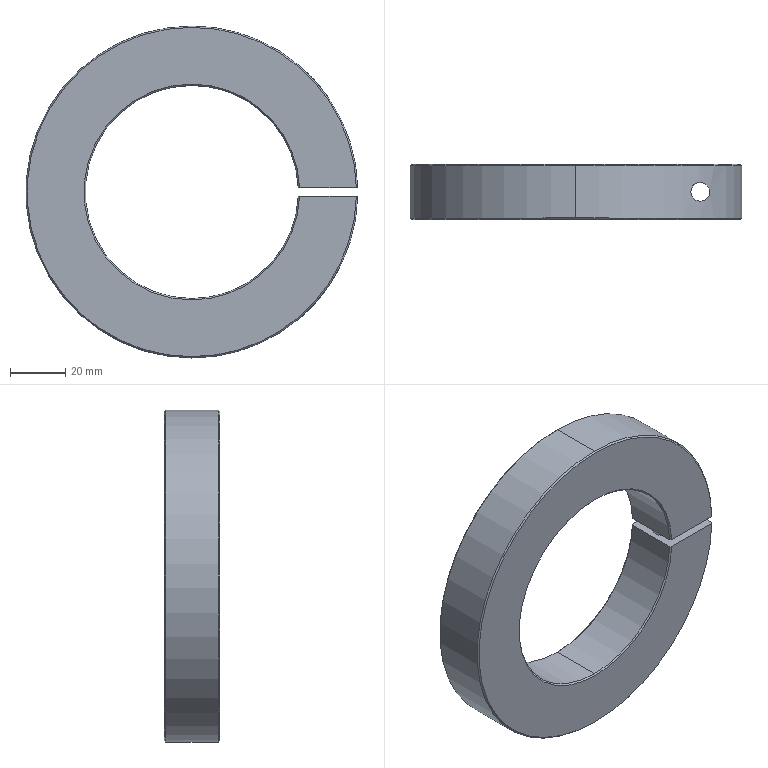Component | SolidWorks | 8TC-A15004-80-18A-1 | 1 solid | 29 faces | box 119.98 x 20 x 120 mm | volume 125088 mm3 | cylinder 12 | cone 12 | plane 5 | commonest cylinder face diameters 77 x3 120 x3 6.8 x2 9 x2 15 x2 | material Black POM
STEP:
#1=COLOUR_RGB('',0.7922,0.8196,0.9333);
#2=FILL_AREA_STYLE_COLOUR('',#1);
#3=FILL_AREA_STYLE('',(#2));
#4=SURFACE_STYLE_FILL_AREA(#3);
#5=SURFACE_SIDE_STYLE('',(#4));
#6=SURFACE_STYLE_USAGE(.BOTH.,#5);
#7=PRESENTATION_STYLE_ASSIGNMENT((#6));
#8=CARTESIAN_POINT('',(3.48,7.618,-28.131));
#9=VERTEX_POINT('',#8);
#10=CARTESIAN_POINT('',(3.213,7.618,-27.825));
#11=VERTEX_POINT('',#10);
#12=CARTESIAN_POINT('',(3.48,7.618,-28.131));
#13=CARTESIAN_POINT('',(3.48,7.613,-28.131));
#14=CARTESIAN_POINT('',(3.48,7.607,-28.131));
#15=CARTESIAN_POINT('',(3.479,7.596,-28.129));
#16=CARTESIAN_POINT('',(3.478,7.591,-28.128));
#17=CARTESIAN_POINT('',(3.475,7.58,-28.124));
#18=CARTESIAN_POINT('',(3.473,7.575,-28.122));
#19=CARTESIAN_POINT('',(3.47,7.566,-28.117));
#20=CARTESIAN_POINT('',(3.468,7.561,-28.115));
#21=CARTESIAN_POINT('',(3.463,7.553,-28.109));
#22=CARTESIAN_POINT('',(3.461,7.549,-28.106));
#23=CARTESIAN_POINT('',(3.456,7.541,-28.099));
#24=CARTESIAN_POINT('',(3.454,7.538,-28.096));
#25=CARTESIAN_POINT('',(3.445,7.528,-28.085));
#26=CARTESIAN_POINT('',(3.44,7.522,-28.078));
#27=CARTESIAN_POINT('',(3.421,7.506,-28.054));
#28=CARTESIAN_POINT('',(3.408,7.498,-28.038));
#29=CARTESIAN_POINT('',(3.388,7.491,-28.013));
#30=CARTESIAN_POINT('',(3.38,7.488,-28.004));
#31=CARTESIAN_POINT('',(3.366,7.486,-27.988));
#32=CARTESIAN_POINT('',(3.359,7.485,-27.979));
#33=CARTESIAN_POINT('',(3.344,7.484,-27.963));
#34=CARTESIAN_POINT('',(3.337,7.484,-27.954));
#35=CARTESIAN_POINT('',(3.322,7.486,-27.938));
#36=CARTESIAN_POINT('',(3.315,7.488,-27.93));
#37=CARTESIAN_POINT('',(3.3,7.492,-27.914));
#38=CARTESIAN_POINT('',(3.292,7.495,-27.906));
#39=CARTESIAN_POINT('',(3.278,7.503,-27.891));
#40=CARTESIAN_POINT('',(3.271,7.507,-27.883));
#41=CARTESIAN_POINT('',(3.257,7.518,-27.869));
#42=CARTESIAN_POINT('',(3.251,7.524,-27.863));
#43=CARTESIAN_POINT('',(3.238,7.538,-27.851));
#44=CARTESIAN_POINT('',(3.233,7.547,-27.845));
#45=CARTESIAN_POINT('',(3.223,7.565,-27.836));
#46=CARTESIAN_POINT('',(3.219,7.575,-27.832));
#47=CARTESIAN_POINT('',(3.214,7.596,-27.827));
#48=CARTESIAN_POINT('',(3.213,7.607,-27.825));
#49=CARTESIAN_POINT('',(3.213,7.618,-27.825));
#50=B_SPLINE_CURVE_WITH_KNOTS('',3,(#12,#13,#14,#15,#16,#17,#18,#19,#20,#21,#22,#23,#24,#25,#26,#27,#28,#29,#30,#31,#32,#33,#34,#35,#36,#37,#38,#39,#40,#41,#42,#43,#44,#45,#46,#47,#48,#49),.UNSPECIFIED.,.F.,.F.,(4,2,2,2,2,2,2,2,2,2,2,2,2,2,2,2,2,2,4),(0.01358,0.014,0.01443,0.01485,0.01527,0.0157,0.01612,0.01697,0.01867,0.01952,0.02037,0.02122,0.02206,0.02291,0.02376,0.02461,0.02546,0.02631,0.02716),.UNSPECIFIED.);
#51=EDGE_CURVE('',#9,#11,#50,.T.);
#52=ORIENTED_EDGE('',*,*,#51,.F.);
#53=CARTESIAN_POINT('',(3.48,7.618,-29.469));
#54=VERTEX_POINT('',#53);
#55=CARTESIAN_POINT('',(3.48,7.618,-29.469));
#56=DIRECTION('',(0.,0.,-1.));
#57=VECTOR('',#56,39.37);
#58=LINE('',#55,#57);
#59=EDGE_CURVE('',#9,#54,#58,.T.);
#60=ORIENTED_EDGE('',*,*,#59,.T.);
#61=CARTESIAN_POINT('',(3.213,7.618,-29.469));
#62=VERTEX_POINT('',#61);
#63=CARTESIAN_POINT('',(3.346,7.618,-29.469));
#64=DIRECTION('',(0.,0.,-1.));
#65=DIRECTION('',(-1.,0.,0.));
#66=AXIS2_PLACEMENT_3D('',#63,#64,#65);
#67=CIRCLE('',#66,0.1339);
#68=EDGE_CURVE('',#54,#62,#67,.T.);
#69=ORIENTED_EDGE('',*,*,#68,.T.);
#70=CARTESIAN_POINT('',(3.213,7.618,-29.469));
#71=DIRECTION('',(0.,0.,-1.));
#72=VECTOR('',#71,39.37);
#73=LINE('',#70,#72);
#74=EDGE_CURVE('',#11,#62,#73,.T.);
#75=ORIENTED_EDGE('',*,*,#74,.F.);
#76=EDGE_LOOP('',(#52,#60,#69,#75));
#77=FACE_OUTER_BOUND('',#76,.T.);
#78=CARTESIAN_POINT('',(3.346,7.618,-29.469));
#79=DIRECTION('',(0.,0.,-1.));
#80=DIRECTION('',(-1.,0.,0.));
#81=AXIS2_PLACEMENT_3D('',#78,#79,#80);
#82=CYLINDRICAL_SURFACE('',#81,0.1339);
#83=ADVANCED_FACE('',(#77),#82,.F.);
#84=CARTESIAN_POINT('',(1.575,7.244,-28.012));
#85=VERTEX_POINT('',#84);
#86=CARTESIAN_POINT('',(1.575,7.244,-31.043));
#87=VERTEX_POINT('',#86);
#88=CARTESIAN_POINT('',(1.575,7.244,-29.528));
#89=DIRECTION('',(0.,-1.,0.));
#90=DIRECTION('',(0.,0.,1.));
#91=AXIS2_PLACEMENT_3D('',#88,#89,#90);
#92=CIRCLE('',#91,1.516);
#93=EDGE_CURVE('',#85,#87,#92,.T.);
#94=ORIENTED_EDGE('',*,*,#93,.F.);
#95=CARTESIAN_POINT('',(1.575,7.224,-27.992));
#96=VERTEX_POINT('',#95);
#97=CARTESIAN_POINT('',(1.575,7.224,-27.992));
#98=DIRECTION('',(0.,-0.7071,0.7071));
#99=VECTOR('',#98,39.37);
#100=LINE('',#97,#99);
#101=EDGE_CURVE('',#85,#96,#100,.T.);
#102=ORIENTED_EDGE('',*,*,#101,.T.);
#103=CARTESIAN_POINT('',(1.575,7.224,-31.063));
#104=VERTEX_POINT('',#103);
#105=CARTESIAN_POINT('',(1.575,7.224,-29.528));
#106=DIRECTION('',(0.,1.,0.));
#107=DIRECTION('',(0.,0.,1.));
#108=AXIS2_PLACEMENT_3D('',#105,#106,#107);
#109=CIRCLE('',#108,1.535);
#110=EDGE_CURVE('',#104,#96,#109,.T.);
#111=ORIENTED_EDGE('',*,*,#110,.F.);
#112=CARTESIAN_POINT('',(1.575,7.224,-31.063));
#113=DIRECTION('',(0.,-0.7071,-0.7071));
#114=VECTOR('',#113,39.37);
#115=LINE('',#112,#114);
#116=EDGE_CURVE('',#87,#104,#115,.T.);
#117=ORIENTED_EDGE('',*,*,#116,.F.);
#118=EDGE_LOOP('',(#94,#102,#111,#117));
#119=FACE_OUTER_BOUND('',#118,.T.);
#120=CARTESIAN_POINT('',(1.575,7.224,-29.528));
#121=DIRECTION('',(0.,-1.,0.));
#122=DIRECTION('',(0.,0.,-1.));
#123=AXIS2_PLACEMENT_3D('',#120,#121,#122);
#124=CONICAL_SURFACE('',#123,1.535,0.7854);
#125=ADVANCED_FACE('',(#119),#124,.F.);
#126=CARTESIAN_POINT('',(3.089,7.244,-29.587));
#127=VERTEX_POINT('',#126);
#128=CARTESIAN_POINT('',(1.575,7.244,-29.528));
#129=DIRECTION('',(0.,-1.,0.));
#130=DIRECTION('',(0.,0.,1.));
#131=AXIS2_PLACEMENT_3D('',#128,#129,#130);
#132=CIRCLE('',#131,1.516);
#133=EDGE_CURVE('',#87,#127,#132,.T.);
#134=ORIENTED_EDGE('',*,*,#133,.F.);
#135=ORIENTED_EDGE('',*,*,#116,.T.);
#136=CARTESIAN_POINT('',(3.109,7.224,-29.587));
#137=VERTEX_POINT('',#136);
#138=CARTESIAN_POINT('',(1.575,7.224,-29.528));
#139=DIRECTION('',(0.,1.,0.));
#140=DIRECTION('',(0.,0.,1.));
#141=AXIS2_PLACEMENT_3D('',#138,#139,#140);
#142=CIRCLE('',#141,1.535);
#143=EDGE_CURVE('',#137,#104,#142,.T.);
#144=ORIENTED_EDGE('',*,*,#143,.F.);
#145=CARTESIAN_POINT('',(3.089,7.244,-29.587));
#146=CARTESIAN_POINT('',(3.096,7.238,-29.587));
#147=CARTESIAN_POINT('',(3.103,7.231,-29.587));
#148=CARTESIAN_POINT('',(3.109,7.224,-29.587));
#149=B_SPLINE_CURVE_WITH_KNOTS('',3,(#145,#146,#147,#148),.UNSPECIFIED.,.F.,.F.,(4,4),(0.,0.0007074),.UNSPECIFIED.);
#150=EDGE_CURVE('',#127,#137,#149,.T.);
#151=ORIENTED_EDGE('',*,*,#150,.F.);
#152=EDGE_LOOP('',(#134,#135,#144,#151));
#153=FACE_OUTER_BOUND('',#152,.T.);
#154=CARTESIAN_POINT('',(1.575,7.224,-29.528));
#155=DIRECTION('',(0.,-1.,0.));
#156=DIRECTION('',(0.,0.,-1.));
#157=AXIS2_PLACEMENT_3D('',#154,#155,#156);
#158=CONICAL_SURFACE('',#157,1.535,0.7854);
#159=ADVANCED_FACE('',(#153),#158,.F.);
#160=CARTESIAN_POINT('',(1.575,7.224,-31.87));
#161=VERTEX_POINT('',#160);
#162=CARTESIAN_POINT('',(3.917,7.224,-29.587));
#163=VERTEX_POINT('',#162);
#164=CARTESIAN_POINT('',(1.575,7.224,-29.528));
#165=DIRECTION('',(0.,-1.,0.));
#166=DIRECTION('',(-0.,0.,1.));
#167=AXIS2_PLACEMENT_3D('',#164,#165,#166);
#168=CIRCLE('',#167,2.343);
#169=EDGE_CURVE('',#161,#163,#168,.T.);
#170=ORIENTED_EDGE('',*,*,#169,.F.);
#171=CARTESIAN_POINT('',(1.575,7.244,-31.89));
#172=VERTEX_POINT('',#171);
#173=CARTESIAN_POINT('',(1.575,7.244,-31.89));
#174=DIRECTION('',(0.,0.7071,-0.7071));
#175=VECTOR('',#174,39.37);
#176=LINE('',#173,#175);
#177=EDGE_CURVE('',#161,#172,#176,.T.);
#178=ORIENTED_EDGE('',*,*,#177,.T.);
#179=CARTESIAN_POINT('',(3.936,7.244,-29.587));
#180=VERTEX_POINT('',#179);
#181=CARTESIAN_POINT('',(1.575,7.244,-29.528));
#182=DIRECTION('',(0.,1.,0.));
#183=DIRECTION('',(0.,0.,1.));
#184=AXIS2_PLACEMENT_3D('',#181,#182,#183);
#185=CIRCLE('',#184,2.362);
#186=EDGE_CURVE('',#180,#172,#185,.T.);
#187=ORIENTED_EDGE('',*,*,#186,.F.);
#188=CARTESIAN_POINT('',(3.917,7.224,-29.587));
#189=CARTESIAN_POINT('',(3.923,7.231,-29.587));
#190=CARTESIAN_POINT('',(3.93,7.238,-29.587));
#191=CARTESIAN_POINT('',(3.936,7.244,-29.587));
#192=B_SPLINE_CURVE_WITH_KNOTS('',3,(#188,#189,#190,#191),.UNSPECIFIED.,.F.,.F.,(4,4),(0.,0.0007072),.UNSPECIFIED.);
#193=EDGE_CURVE('',#163,#180,#192,.T.);
#194=ORIENTED_EDGE('',*,*,#193,.F.);
#195=EDGE_LOOP('',(#170,#178,#187,#194));
#196=FACE_OUTER_BOUND('',#195,.T.);
#197=CARTESIAN_POINT('',(1.575,7.244,-29.528));
#198=DIRECTION('',(0.,1.,0.));
#199=DIRECTION('',(0.,0.,1.));
#200=AXIS2_PLACEMENT_3D('',#197,#198,#199);
#201=CONICAL_SURFACE('',#200,2.362,0.7854);
#202=ADVANCED_FACE('',(#196),#201,.T.);
#203=ORIENTED_EDGE('',*,*,#177,.F.);
#204=CARTESIAN_POINT('',(1.575,7.224,-27.185));
#205=VERTEX_POINT('',#204);
#206=CARTESIAN_POINT('',(1.575,7.224,-29.528));
#207=DIRECTION('',(0.,-1.,0.));
#208=DIRECTION('',(0.,0.,1.));
#209=AXIS2_PLACEMENT_3D('',#206,#207,#208);
#210=CIRCLE('',#209,2.343);
#211=EDGE_CURVE('',#205,#161,#210,.T.);
#212=ORIENTED_EDGE('',*,*,#211,.F.);
#213=CARTESIAN_POINT('',(1.575,7.244,-27.165));
#214=VERTEX_POINT('',#213);
#215=CARTESIAN_POINT('',(1.575,7.244,-27.165));
#216=DIRECTION('',(0.,0.7071,0.7071));
#217=VECTOR('',#216,39.37);
#218=LINE('',#215,#217);
#219=EDGE_CURVE('',#205,#214,#218,.T.);
#220=ORIENTED_EDGE('',*,*,#219,.T.);
#221=CARTESIAN_POINT('',(1.575,7.244,-29.528));
#222=DIRECTION('',(0.,1.,0.));
#223=DIRECTION('',(0.,0.,1.));
#224=AXIS2_PLACEMENT_3D('',#221,#222,#223);
#225=CIRCLE('',#224,2.362);
#226=EDGE_CURVE('',#172,#214,#225,.T.);
#227=ORIENTED_EDGE('',*,*,#226,.F.);
#228=EDGE_LOOP('',(#203,#212,#220,#227));
#229=FACE_OUTER_BOUND('',#228,.T.);
#230=CARTESIAN_POINT('',(1.575,7.244,-29.528));
#231=DIRECTION('',(0.,1.,0.));
#232=DIRECTION('',(0.,0.,1.));
#233=AXIS2_PLACEMENT_3D('',#230,#231,#232);
#234=CONICAL_SURFACE('',#233,2.362,0.7854);
#235=ADVANCED_FACE('',(#229),#234,.T.);
#236=CARTESIAN_POINT('',(1.575,8.012,-27.185));
#237=VERTEX_POINT('',#236);
#238=CARTESIAN_POINT('',(3.917,8.012,-29.469));
#239=VERTEX_POINT('',#238);
#240=CARTESIAN_POINT('',(1.575,8.012,-29.528));
#241=DIRECTION('',(0.,1.,0.));
#242=DIRECTION('',(0.,0.,1.));
#243=AXIS2_PLACEMENT_3D('',#240,#241,#242);
#244=CIRCLE('',#243,2.343);
#245=EDGE_CURVE('',#237,#239,#244,.T.);
#246=ORIENTED_EDGE('',*,*,#245,.F.);
#247=CARTESIAN_POINT('',(1.575,7.992,-27.165));
#248=VERTEX_POINT('',#247);
#249=CARTESIAN_POINT('',(1.575,8.012,-27.185));
#250=DIRECTION('',(0.,-0.7071,0.7071));
#251=VECTOR('',#250,39.37);
#252=LINE('',#249,#251);
#253=EDGE_CURVE('',#237,#248,#252,.T.);
#254=ORIENTED_EDGE('',*,*,#253,.T.);
#255=CARTESIAN_POINT('',(3.936,7.992,-29.469));
#256=VERTEX_POINT('',#255);
#257=CARTESIAN_POINT('',(1.575,7.992,-29.528));
#258=DIRECTION('',(0.,-1.,0.));
#259=DIRECTION('',(-0.,0.,1.));
#260=AXIS2_PLACEMENT_3D('',#257,#258,#259);
#261=CIRCLE('',#260,2.362);
#262=EDGE_CURVE('',#256,#248,#261,.T.);
#263=ORIENTED_EDGE('',*,*,#262,.F.);
#264=CARTESIAN_POINT('',(3.917,8.012,-29.469));
#265=CARTESIAN_POINT('',(3.923,8.005,-29.469));
#266=CARTESIAN_POINT('',(3.93,7.999,-29.469));
#267=CARTESIAN_POINT('',(3.936,7.992,-29.469));
#268=B_SPLINE_CURVE_WITH_KNOTS('',3,(#264,#265,#266,#267),.UNSPECIFIED.,.F.,.F.,(4,4),(0.,0.0007072),.UNSPECIFIED.);
#269=EDGE_CURVE('',#239,#256,#268,.T.);
#270=ORIENTED_EDGE('',*,*,#269,.F.);
#271=EDGE_LOOP('',(#246,#254,#263,#270));
#272=FACE_OUTER_BOUND('',#271,.T.);
#273=CARTESIAN_POINT('',(1.575,8.012,-29.528));
#274=DIRECTION('',(0.,-1.,0.));
#275=DIRECTION('',(0.,0.,-1.));
#276=AXIS2_PLACEMENT_3D('',#273,#274,#275);
#277=CONICAL_SURFACE('',#276,2.343,0.7854);
#278=ADVANCED_FACE('',(#272),#277,.T.);
#279=ORIENTED_EDGE('',*,*,#253,.F.);
#280=CARTESIAN_POINT('',(1.575,8.012,-31.87));
#281=VERTEX_POINT('',#280);
#282=CARTESIAN_POINT('',(1.575,8.012,-29.528));
#283=DIRECTION('',(0.,1.,0.));
#284=DIRECTION('',(0.,0.,1.));
#285=AXIS2_PLACEMENT_3D('',#282,#283,#284);
#286=CIRCLE('',#285,2.343);
#287=EDGE_CURVE('',#281,#237,#286,.T.);
#288=ORIENTED_EDGE('',*,*,#287,.F.);
#289=CARTESIAN_POINT('',(1.575,7.992,-31.89));
#290=VERTEX_POINT('',#289);
#291=CARTESIAN_POINT('',(1.575,8.012,-31.87));
#292=DIRECTION('',(0.,-0.7071,-0.7071));
#293=VECTOR('',#292,39.37);
#294=LINE('',#291,#293);
#295=EDGE_CURVE('',#281,#290,#294,.T.);
#296=ORIENTED_EDGE('',*,*,#295,.T.);
#297=CARTESIAN_POINT('',(1.575,7.992,-29.528));
#298=DIRECTION('',(0.,-1.,0.));
#299=DIRECTION('',(0.,0.,1.));
#300=AXIS2_PLACEMENT_3D('',#297,#298,#299);
#301=CIRCLE('',#300,2.362);
#302=EDGE_CURVE('',#248,#290,#301,.T.);
#303=ORIENTED_EDGE('',*,*,#302,.F.);
#304=EDGE_LOOP('',(#279,#288,#296,#303));
#305=FACE_OUTER_BOUND('',#304,.T.);
#306=CARTESIAN_POINT('',(1.575,8.012,-29.528));
#307=DIRECTION('',(0.,-1.,0.));
#308=DIRECTION('',(0.,0.,-1.));
#309=AXIS2_PLACEMENT_3D('',#306,#307,#308);
#310=CONICAL_SURFACE('',#309,2.343,0.7854);
#311=ADVANCED_FACE('',(#305),#310,.T.);
#312=CARTESIAN_POINT('',(1.575,7.992,-31.043));
#313=VERTEX_POINT('',#312);
#314=CARTESIAN_POINT('',(1.575,7.992,-28.012));
#315=VERTEX_POINT('',#314);
#316=CARTESIAN_POINT('',(1.575,7.992,-29.528));
#317=DIRECTION('',(0.,1.,0.));
#318=DIRECTION('',(0.,0.,1.));
#319=AXIS2_PLACEMENT_3D('',#316,#317,#318);
#320=CIRCLE('',#319,1.516);
#321=EDGE_CURVE('',#313,#315,#320,.T.);
#322=ORIENTED_EDGE('',*,*,#321,.F.);
#323=CARTESIAN_POINT('',(1.575,8.012,-31.063));
#324=VERTEX_POINT('',#323);
#325=CARTESIAN_POINT('',(1.575,7.992,-31.043));
#326=DIRECTION('',(0.,0.7071,-0.7071));
#327=VECTOR('',#326,39.37);
#328=LINE('',#325,#327);
#329=EDGE_CURVE('',#313,#324,#328,.T.);
#330=ORIENTED_EDGE('',*,*,#329,.T.);
#331=CARTESIAN_POINT('',(1.575,8.012,-27.992));
#332=VERTEX_POINT('',#331);
#333=CARTESIAN_POINT('',(1.575,8.012,-29.528));
#334=DIRECTION('',(0.,-1.,0.));
#335=DIRECTION('',(0.,0.,1.));
#336=AXIS2_PLACEMENT_3D('',#333,#334,#335);
#337=CIRCLE('',#336,1.535);
#338=EDGE_CURVE('',#332,#324,#337,.T.);
#339=ORIENTED_EDGE('',*,*,#338,.F.);
#340=CARTESIAN_POINT('',(1.575,7.992,-28.012));
#341=DIRECTION('',(0.,0.7071,0.7071));
#342=VECTOR('',#341,39.37);
#343=LINE('',#340,#342);
#344=EDGE_CURVE('',#315,#332,#343,.T.);
#345=ORIENTED_EDGE('',*,*,#344,.F.);
#346=EDGE_LOOP('',(#322,#330,#339,#345));
#347=FACE_OUTER_BOUND('',#346,.T.);
#348=CARTESIAN_POINT('',(1.575,7.992,-29.528));
#349=DIRECTION('',(0.,1.,0.));
#350=DIRECTION('',(0.,0.,1.));
#351=AXIS2_PLACEMENT_3D('',#348,#349,#350);
#352=CONICAL_SURFACE('',#351,1.516,0.7854);
#353=ADVANCED_FACE('',(#347),#352,.F.);
#354=CARTESIAN_POINT('',(3.089,7.992,-29.469));
#355=VERTEX_POINT('',#354);
#356=CARTESIAN_POINT('',(1.575,7.992,-29.528));
#357=DIRECTION('',(0.,1.,0.));
#358=DIRECTION('',(0.,0.,1.));
#359=AXIS2_PLACEMENT_3D('',#356,#357,#358);
#360=CIRCLE('',#359,1.516);
#361=EDGE_CURVE('',#315,#355,#360,.T.);
#362=ORIENTED_EDGE('',*,*,#361,.F.);
#363=ORIENTED_EDGE('',*,*,#344,.T.);
#364=CARTESIAN_POINT('',(3.109,8.012,-29.469));
#365=VERTEX_POINT('',#364);
#366=CARTESIAN_POINT('',(1.575,8.012,-29.528));
#367=DIRECTION('',(0.,-1.,0.));
#368=DIRECTION('',(-0.,0.,1.));
#369=AXIS2_PLACEMENT_3D('',#366,#367,#368);
#370=CIRCLE('',#369,1.535);
#371=EDGE_CURVE('',#365,#332,#370,.T.);
#372=ORIENTED_EDGE('',*,*,#371,.F.);
#373=CARTESIAN_POINT('',(3.089,7.992,-29.469));
#374=CARTESIAN_POINT('',(3.096,7.999,-29.469));
#375=CARTESIAN_POINT('',(3.103,8.005,-29.469));
#376=CARTESIAN_POINT('',(3.109,8.012,-29.469));
#377=B_SPLINE_CURVE_WITH_KNOTS('',3,(#373,#374,#375,#376),.UNSPECIFIED.,.F.,.F.,(4,4),(0.,0.0007074),.UNSPECIFIED.);
#378=EDGE_CURVE('',#355,#365,#377,.T.);
#379=ORIENTED_EDGE('',*,*,#378,.F.);
#380=EDGE_LOOP('',(#362,#363,#372,#379));
#381=FACE_OUTER_BOUND('',#380,.T.);
#382=CARTESIAN_POINT('',(1.575,7.992,-29.528));
#383=DIRECTION('',(0.,1.,0.));
#384=DIRECTION('',(0.,0.,1.));
#385=AXIS2_PLACEMENT_3D('',#382,#383,#384);
#386=CONICAL_SURFACE('',#385,1.516,0.7854);
#387=ADVANCED_FACE('',(#381),#386,.F.);
#388=CARTESIAN_POINT('',(3.169,7.618,-29.587));
#389=VERTEX_POINT('',#388);
#390=CARTESIAN_POINT('',(3.524,7.618,-29.587));
#391=VERTEX_POINT('',#390);
#392=CARTESIAN_POINT('',(3.346,7.618,-29.587));
#393=DIRECTION('',(-0.,0.,1.));
#394=DIRECTION('',(-1.,0.,0.));
#395=AXIS2_PLACEMENT_3D('',#392,#393,#394);
#396=CIRCLE('',#395,0.1772);
#397=EDGE_CURVE('',#389,#391,#396,.T.);
#398=ORIENTED_EDGE('',*,*,#397,.T.);
#399=CARTESIAN_POINT('',(3.524,7.618,-30.118));
#400=VERTEX_POINT('',#399);
#401=CARTESIAN_POINT('',(3.524,7.618,-31.496));
#402=DIRECTION('',(0.,0.,-1.));
#403=VECTOR('',#402,39.37);
#404=LINE('',#401,#403);
#405=EDGE_CURVE('',#391,#400,#404,.T.);
#406=ORIENTED_EDGE('',*,*,#405,.T.);
#407=CARTESIAN_POINT('',(3.169,7.618,-30.118));
#408=VERTEX_POINT('',#407);
#409=CARTESIAN_POINT('',(3.346,7.618,-30.118));
#410=DIRECTION('',(0.,0.,-1.));
#411=DIRECTION('',(-1.,0.,0.));
#412=AXIS2_PLACEMENT_3D('',#409,#410,#411);
#413=CIRCLE('',#412,0.1772);
#414=EDGE_CURVE('',#400,#408,#413,.T.);
#415=ORIENTED_EDGE('',*,*,#414,.T.);
#416=CARTESIAN_POINT('',(3.169,7.618,-31.496));
#417=DIRECTION('',(0.,0.,-1.));
#418=VECTOR('',#417,39.37);
#419=LINE('',#416,#418);
#420=EDGE_CURVE('',#389,#408,#419,.T.);
#421=ORIENTED_EDGE('',*,*,#420,.F.);
#422=EDGE_LOOP('',(#398,#406,#415,#421));
#423=FACE_OUTER_BOUND('',#422,.T.);
#424=CARTESIAN_POINT('',(3.346,7.618,-31.496));
#425=DIRECTION('',(0.,0.,-1.));
#426=DIRECTION('',(-1.,0.,0.));
#427=AXIS2_PLACEMENT_3D('',#424,#425,#426);
#428=CYLINDRICAL_SURFACE('',#427,0.1772);
#429=ADVANCED_FACE('',(#423),#428,.F.);
#430=CARTESIAN_POINT('',(3.642,7.618,-30.118));
#431=VERTEX_POINT('',#430);
#432=CARTESIAN_POINT('',(3.051,7.618,-30.118));
#433=VERTEX_POINT('',#432);
#434=CARTESIAN_POINT('',(3.346,7.618,-30.118));
#435=DIRECTION('',(0.,0.,-1.));
#436=DIRECTION('',(-1.,0.,0.));
#437=AXIS2_PLACEMENT_3D('',#434,#435,#436);
#438=CIRCLE('',#437,0.2953);
#439=EDGE_CURVE('',#431,#433,#438,.T.);
#440=ORIENTED_EDGE('',*,*,#439,.F.);
#441=CARTESIAN_POINT('',(3.642,7.618,-30.671));
#442=VERTEX_POINT('',#441);
#443=CARTESIAN_POINT('',(3.642,7.618,-31.496));
#444=DIRECTION('',(0.,0.,-1.));
#445=VECTOR('',#444,39.37);
#446=LINE('',#443,#445);
#447=EDGE_CURVE('',#431,#442,#446,.T.);
#448=ORIENTED_EDGE('',*,*,#447,.T.);
#449=CARTESIAN_POINT('',(3.051,7.618,-31.372));
#450=VERTEX_POINT('',#449);
#451=CARTESIAN_POINT('',(3.051,7.618,-31.372));
#452=CARTESIAN_POINT('',(3.051,7.593,-31.372));
#453=CARTESIAN_POINT('',(3.054,7.568,-31.369));
#454=CARTESIAN_POINT('',(3.064,7.532,-31.361));
#455=CARTESIAN_POINT('',(3.067,7.521,-31.358));
#456=CARTESIAN_POINT('',(3.076,7.498,-31.351));
#457=CARTESIAN_POINT('',(3.081,7.488,-31.347));
#458=CARTESIAN_POINT('',(3.092,7.467,-31.338));
#459=CARTESIAN_POINT('',(3.099,7.457,-31.333));
#460=CARTESIAN_POINT('',(3.112,7.439,-31.322));
#461=CARTESIAN_POINT('',(3.118,7.43,-31.316));
#462=CARTESIAN_POINT('',(3.133,7.414,-31.303));
#463=CARTESIAN_POINT('',(3.14,7.406,-31.296));
#464=CARTESIAN_POINT('',(3.156,7.392,-31.283));
#465=CARTESIAN_POINT('',(3.164,7.386,-31.275));
#466=CARTESIAN_POINT('',(3.188,7.368,-31.253));
#467=CARTESIAN_POINT('',(3.205,7.358,-31.237));
#468=CARTESIAN_POINT('',(3.23,7.346,-31.213));
#469=CARTESIAN_POINT('',(3.239,7.343,-31.204));
#470=CARTESIAN_POINT('',(3.256,7.337,-31.187));
#471=CARTESIAN_POINT('',(3.265,7.334,-31.178));
#472=CARTESIAN_POINT('',(3.29,7.328,-31.152));
#473=CARTESIAN_POINT('',(3.307,7.325,-31.134));
#474=CARTESIAN_POINT('',(3.341,7.322,-31.097));
#475=CARTESIAN_POINT('',(3.357,7.323,-31.078));
#476=CARTESIAN_POINT('',(3.406,7.327,-31.021));
#477=CARTESIAN_POINT('',(3.436,7.335,-30.983));
#478=CARTESIAN_POINT('',(3.479,7.354,-30.925));
#479=CARTESIAN_POINT('',(3.493,7.361,-30.906));
#480=CARTESIAN_POINT('',(3.52,7.379,-30.867));
#481=CARTESIAN_POINT('',(3.533,7.389,-30.849));
#482=CARTESIAN_POINT('',(3.558,7.411,-30.811));
#483=CARTESIAN_POINT('',(3.569,7.424,-30.793));
#484=CARTESIAN_POINT('',(3.586,7.445,-30.767));
#485=CARTESIAN_POINT('',(3.591,7.452,-30.758));
#486=CARTESIAN_POINT('',(3.601,7.468,-30.742));
#487=CARTESIAN_POINT('',(3.606,7.477,-30.734));
#488=CARTESIAN_POINT('',(3.615,7.495,-30.719));
#489=CARTESIAN_POINT('',(3.619,7.504,-30.711));
#490=CARTESIAN_POINT('',(3.627,7.524,-30.698));
#491=CARTESIAN_POINT('',(3.63,7.535,-30.692));
#492=CARTESIAN_POINT('',(3.636,7.557,-30.682));
#493=CARTESIAN_POINT('',(3.638,7.569,-30.678));
#494=CARTESIAN_POINT('',(3.64,7.587,-30.674));
#495=CARTESIAN_POINT('',(3.641,7.593,-30.673));
#496=CARTESIAN_POINT('',(3.642,7.605,-30.672));
#497=CARTESIAN_POINT('',(3.642,7.612,-30.671));
#498=CARTESIAN_POINT('',(3.642,7.618,-30.671));
#499=B_SPLINE_CURVE_WITH_KNOTS('',3,(#451,#452,#453,#454,#455,#456,#457,#458,#459,#460,#461,#462,#463,#464,#465,#466,#467,#468,#469,#470,#471,#472,#473,#474,#475,#476,#477,#478,#479,#480,#481,#482,#483,#484,#485,#486,#487,#488,#489,#490,#491,#492,#493,#494,#495,#496,#497,#498),.UNSPECIFIED.,.F.,.F.,(4,2,2,2,2,2,2,2,2,2,2,2,2,2,2,2,2,2,2,2,2,2,2,4),(0.,0.001901,0.002851,0.003801,0.004752,0.005702,0.006653,0.007603,0.009504,0.01045,0.0114,0.01331,0.01521,0.01901,0.02091,0.02281,0.02471,0.02566,0.02661,0.02756,0.02851,0.02946,0.02994,0.03041),.UNSPECIFIED.);
#500=EDGE_CURVE('',#450,#442,#499,.T.);
#501=ORIENTED_EDGE('',*,*,#500,.F.);
#502=CARTESIAN_POINT('',(3.051,7.618,-31.496));
#503=DIRECTION('',(0.,0.,-1.));
#504=VECTOR('',#503,39.37);
#505=LINE('',#502,#504);
#506=EDGE_CURVE('',#433,#450,#505,.T.);
#507=ORIENTED_EDGE('',*,*,#506,.F.);
#508=EDGE_LOOP('',(#440,#448,#501,#507));
#509=FACE_OUTER_BOUND('',#508,.T.);
#510=CARTESIAN_POINT('',(3.346,7.618,-31.496));
#511=DIRECTION('',(0.,0.,-1.));
#512=DIRECTION('',(-1.,0.,0.));
#513=AXIS2_PLACEMENT_3D('',#510,#511,#512);
#514=CYLINDRICAL_SURFACE('',#513,0.2953);
#515=ADVANCED_FACE('',(#509),#514,.F.);
#516=ORIENTED_EDGE('',*,*,#321,.T.);
#517=CARTESIAN_POINT('',(1.575,8.012,-28.012));
#518=DIRECTION('',(0.,-1.,0.));
#519=VECTOR('',#518,39.37);
#520=LINE('',#517,#519);
#521=EDGE_CURVE('',#315,#85,#520,.T.);
#522=ORIENTED_EDGE('',*,*,#521,.T.);
#523=ORIENTED_EDGE('',*,*,#93,.T.);
#524=CARTESIAN_POINT('',(1.575,8.012,-31.043));
#525=DIRECTION('',(0.,-1.,0.));
#526=VECTOR('',#525,39.37);
#527=LINE('',#524,#526);
#528=EDGE_CURVE('',#313,#87,#527,.T.);
#529=ORIENTED_EDGE('',*,*,#528,.F.);
#530=EDGE_LOOP('',(#516,#522,#523,#529));
#531=FACE_OUTER_BOUND('',#530,.T.);
#532=CARTESIAN_POINT('',(1.575,8.012,-29.528));
#533=DIRECTION('',(0.,-1.,0.));
#534=DIRECTION('',(0.,0.,-1.));
#535=AXIS2_PLACEMENT_3D('',#532,#533,#534);
#536=CYLINDRICAL_SURFACE('',#535,1.516);
#537=ADVANCED_FACE('',(#531),#536,.F.);
#538=CARTESIAN_POINT('',(3.089,7.992,-29.587));
#539=VERTEX_POINT('',#538);
#540=CARTESIAN_POINT('',(1.575,7.992,-29.528));
#541=DIRECTION('',(0.,1.,0.));
#542=DIRECTION('',(0.,0.,1.));
#543=AXIS2_PLACEMENT_3D('',#540,#541,#542);
#544=CIRCLE('',#543,1.516);
#545=EDGE_CURVE('',#539,#313,#544,.T.);
#546=ORIENTED_EDGE('',*,*,#545,.T.);
#547=ORIENTED_EDGE('',*,*,#528,.T.);
#548=ORIENTED_EDGE('',*,*,#133,.T.);
#549=CARTESIAN_POINT('',(3.089,7.224,-29.587));
#550=DIRECTION('',(0.,1.,0.));
#551=VECTOR('',#550,39.37);
#552=LINE('',#549,#551);
#553=EDGE_CURVE('',#127,#539,#552,.T.);
#554=ORIENTED_EDGE('',*,*,#553,.T.);
#555=EDGE_LOOP('',(#546,#547,#548,#554));
#556=FACE_OUTER_BOUND('',#555,.T.);
#557=CARTESIAN_POINT('',(1.575,8.012,-29.528));
#558=DIRECTION('',(0.,-1.,0.));
#559=DIRECTION('',(0.,0.,-1.));
#560=AXIS2_PLACEMENT_3D('',#557,#558,#559);
#561=CYLINDRICAL_SURFACE('',#560,1.516);
#562=ADVANCED_FACE('',(#556),#561,.F.);
#563=CARTESIAN_POINT('',(3.213,7.618,-27.825));
#564=CARTESIAN_POINT('',(3.213,7.629,-27.825));
#565=CARTESIAN_POINT('',(3.214,7.64,-27.827));
#566=CARTESIAN_POINT('',(3.219,7.662,-27.832));
#567=CARTESIAN_POINT('',(3.223,7.672,-27.836));
#568=CARTESIAN_POINT('',(3.233,7.69,-27.845));
#569=CARTESIAN_POINT('',(3.238,7.698,-27.851));
#570=CARTESIAN_POINT('',(3.251,7.712,-27.863));
#571=CARTESIAN_POINT('',(3.257,7.718,-27.869));
#572=CARTESIAN_POINT('',(3.271,7.729,-27.883));
#573=CARTESIAN_POINT('',(3.278,7.733,-27.891));
#574=CARTESIAN_POINT('',(3.292,7.741,-27.906));
#575=CARTESIAN_POINT('',(3.3,7.744,-27.914));
#576=CARTESIAN_POINT('',(3.322,7.751,-27.938));
#577=CARTESIAN_POINT('',(3.337,7.752,-27.954));
#578=CARTESIAN_POINT('',(3.359,7.752,-27.979));
#579=CARTESIAN_POINT('',(3.366,7.751,-27.988));
#580=CARTESIAN_POINT('',(3.381,7.748,-28.005));
#581=CARTESIAN_POINT('',(3.388,7.746,-28.013));
#582=CARTESIAN_POINT('',(3.401,7.74,-28.029));
#583=CARTESIAN_POINT('',(3.408,7.737,-28.038));
#584=CARTESIAN_POINT('',(3.421,7.73,-28.054));
#585=CARTESIAN_POINT('',(3.427,7.725,-28.062));
#586=CARTESIAN_POINT('',(3.44,7.715,-28.078));
#587=CARTESIAN_POINT('',(3.445,7.709,-28.085));
#588=CARTESIAN_POINT('',(3.456,7.695,-28.099));
#589=CARTESIAN_POINT('',(3.461,7.688,-28.106));
#590=CARTESIAN_POINT('',(3.47,7.671,-28.117));
#591=CARTESIAN_POINT('',(3.474,7.661,-28.122));
#592=CARTESIAN_POINT('',(3.478,7.646,-28.128));
#593=CARTESIAN_POINT('',(3.479,7.64,-28.129));
#594=CARTESIAN_POINT('',(3.48,7.629,-28.131));
#595=CARTESIAN_POINT('',(3.48,7.624,-28.131));
#596=CARTESIAN_POINT('',(3.48,7.618,-28.131));
#597=B_SPLINE_CURVE_WITH_KNOTS('',3,(#563,#564,#565,#566,#567,#568,#569,#570,#571,#572,#573,#574,#575,#576,#577,#578,#579,#580,#581,#582,#583,#584,#585,#586,#587,#588,#589,#590,#591,#592,#593,#594,#595,#596),.UNSPECIFIED.,.F.,.F.,(4,2,2,2,2,2,2,2,2,2,2,2,2,2,2,2,4),(0.,0.0008486,0.001697,0.002546,0.003394,0.004243,0.005091,0.006789,0.007637,0.008486,0.009334,0.01018,0.01103,0.01188,0.01273,0.01315,0.01358),.UNSPECIFIED.);
#598=EDGE_CURVE('',#11,#9,#597,.T.);
#599=ORIENTED_EDGE('',*,*,#598,.T.);
#600=ORIENTED_EDGE('',*,*,#51,.T.);
#601=EDGE_LOOP('',(#599,#600));
#602=FACE_BOUND('',#601,.T.);
#603=ORIENTED_EDGE('',*,*,#262,.T.);
#604=CARTESIAN_POINT('',(1.575,8.012,-27.165));
#605=DIRECTION('',(0.,-1.,0.));
#606=VECTOR('',#605,39.37);
#607=LINE('',#604,#606);
#608=EDGE_CURVE('',#248,#214,#607,.T.);
#609=ORIENTED_EDGE('',*,*,#608,.T.);
#610=CARTESIAN_POINT('',(3.936,7.244,-29.469));
#611=VERTEX_POINT('',#610);
#612=CARTESIAN_POINT('',(1.575,7.244,-29.528));
#613=DIRECTION('',(0.,1.,0.));
#614=DIRECTION('',(0.,0.,1.));
#615=AXIS2_PLACEMENT_3D('',#612,#613,#614);
#616=CIRCLE('',#615,2.362);
#617=EDGE_CURVE('',#214,#611,#616,.T.);
#618=ORIENTED_EDGE('',*,*,#617,.T.);
#619=CARTESIAN_POINT('',(3.936,8.012,-29.469));
#620=DIRECTION('',(0.,1.,0.));
#621=VECTOR('',#620,39.37);
#622=LINE('',#619,#621);
#623=EDGE_CURVE('',#611,#256,#622,.T.);
#624=ORIENTED_EDGE('',*,*,#623,.T.);
#625=EDGE_LOOP('',(#603,#609,#618,#624));
#626=FACE_OUTER_BOUND('',#625,.T.);
#627=CARTESIAN_POINT('',(1.575,8.012,-29.528));
#628=DIRECTION('',(0.,-1.,0.));
#629=DIRECTION('',(0.,0.,-1.));
#630=AXIS2_PLACEMENT_3D('',#627,#628,#629);
#631=CYLINDRICAL_SURFACE('',#630,2.362);
#632=ADVANCED_FACE('',(#602,#626),#631,.T.);
#633=ORIENTED_EDGE('',*,*,#608,.F.);
#634=ORIENTED_EDGE('',*,*,#302,.T.);
#635=CARTESIAN_POINT('',(1.575,8.012,-31.89));
#636=DIRECTION('',(0.,-1.,0.));
#637=VECTOR('',#636,39.37);
#638=LINE('',#635,#637);
#639=EDGE_CURVE('',#290,#172,#638,.T.);
#640=ORIENTED_EDGE('',*,*,#639,.T.);
#641=ORIENTED_EDGE('',*,*,#226,.T.);
#642=EDGE_LOOP('',(#633,#634,#640,#641));
#643=FACE_OUTER_BOUND('',#642,.T.);
#644=CARTESIAN_POINT('',(1.575,8.012,-29.528));
#645=DIRECTION('',(0.,-1.,0.));
#646=DIRECTION('',(0.,0.,-1.));
#647=AXIS2_PLACEMENT_3D('',#644,#645,#646);
#648=CYLINDRICAL_SURFACE('',#647,2.362);
#649=ADVANCED_FACE('',(#643),#648,.T.);
#650=CARTESIAN_POINT('',(3.089,7.244,-29.469));
#651=VERTEX_POINT('',#650);
#652=CARTESIAN_POINT('',(3.089,7.224,-29.469));
#653=DIRECTION('',(0.,1.,0.));
#654=VECTOR('',#653,39.37);
#655=LINE('',#652,#654);
#656=EDGE_CURVE('',#651,#355,#655,.T.);
#657=ORIENTED_EDGE('',*,*,#656,.T.);
#658=ORIENTED_EDGE('',*,*,#378,.T.);
#659=CARTESIAN_POINT('',(3.089,8.012,-29.469));
#660=DIRECTION('',(1.,0.,0.));
#661=VECTOR('',#660,39.37);
#662=LINE('',#659,#661);
#663=EDGE_CURVE('',#365,#239,#662,.T.);
#664=ORIENTED_EDGE('',*,*,#663,.T.);
#665=ORIENTED_EDGE('',*,*,#269,.T.);
#666=ORIENTED_EDGE('',*,*,#623,.F.);
#667=CARTESIAN_POINT('',(3.917,7.224,-29.469));
#668=VERTEX_POINT('',#667);
#669=CARTESIAN_POINT('',(3.936,7.244,-29.469));
#670=CARTESIAN_POINT('',(3.93,7.238,-29.469));
#671=CARTESIAN_POINT('',(3.923,7.231,-29.469));
#672=CARTESIAN_POINT('',(3.917,7.224,-29.469));
#673=B_SPLINE_CURVE_WITH_KNOTS('',3,(#669,#670,#671,#672),.UNSPECIFIED.,.F.,.F.,(4,4),(0.,0.0007072),.UNSPECIFIED.);
#674=EDGE_CURVE('',#611,#668,#673,.T.);
#675=ORIENTED_EDGE('',*,*,#674,.T.);
#676=CARTESIAN_POINT('',(3.109,7.224,-29.469));
#677=VERTEX_POINT('',#676);
#678=CARTESIAN_POINT('',(3.089,7.224,-29.469));
#679=DIRECTION('',(1.,0.,0.));
#680=VECTOR('',#679,39.37);
#681=LINE('',#678,#680);
#682=EDGE_CURVE('',#677,#668,#681,.T.);
#683=ORIENTED_EDGE('',*,*,#682,.F.);
#684=CARTESIAN_POINT('',(3.109,7.224,-29.469));
#685=CARTESIAN_POINT('',(3.103,7.231,-29.469));
#686=CARTESIAN_POINT('',(3.096,7.238,-29.469));
#687=CARTESIAN_POINT('',(3.089,7.244,-29.469));
#688=B_SPLINE_CURVE_WITH_KNOTS('',3,(#684,#685,#686,#687),.UNSPECIFIED.,.F.,.F.,(4,4),(0.,0.0007074),.UNSPECIFIED.);
#689=EDGE_CURVE('',#677,#651,#688,.T.);
#690=ORIENTED_EDGE('',*,*,#689,.T.);
#691=EDGE_LOOP('',(#657,#658,#664,#665,#666,#675,#683,#690));
#692=FACE_OUTER_BOUND('',#691,.T.);
#693=CARTESIAN_POINT('',(3.346,7.618,-29.469));
#694=DIRECTION('',(0.,0.,-1.));
#695=DIRECTION('',(-1.,0.,0.));
#696=AXIS2_PLACEMENT_3D('',#693,#694,#695);
#697=CIRCLE('',#696,0.1339);
#698=EDGE_CURVE('',#62,#54,#697,.T.);
#699=ORIENTED_EDGE('',*,*,#698,.F.);
#700=ORIENTED_EDGE('',*,*,#68,.F.);
#701=EDGE_LOOP('',(#699,#700));
#702=FACE_BOUND('',#701,.T.);
#703=CARTESIAN_POINT('',(3.089,7.224,-29.469));
#704=DIRECTION('',(-0.,0.,1.));
#705=DIRECTION('',(1.,0.,0.));
#706=AXIS2_PLACEMENT_3D('',#703,#704,#705);
#707=PLANE('',#706);
#708=ADVANCED_FACE('',(#692,#702),#707,.F.);
#709=ORIENTED_EDGE('',*,*,#663,.F.);
#710=ORIENTED_EDGE('',*,*,#371,.T.);
#711=ORIENTED_EDGE('',*,*,#338,.T.);
#712=CARTESIAN_POINT('',(3.109,8.012,-29.587));
#713=VERTEX_POINT('',#712);
#714=CARTESIAN_POINT('',(1.575,8.012,-29.528));
#715=DIRECTION('',(0.,-1.,0.));
#716=DIRECTION('',(0.,0.,1.));
#717=AXIS2_PLACEMENT_3D('',#714,#715,#716);
#718=CIRCLE('',#717,1.535);
#719=EDGE_CURVE('',#324,#713,#718,.T.);
#720=ORIENTED_EDGE('',*,*,#719,.T.);
#721=CARTESIAN_POINT('',(3.917,8.012,-29.587));
#722=VERTEX_POINT('',#721);
#723=CARTESIAN_POINT('',(3.089,8.012,-29.587));
#724=DIRECTION('',(-1.,0.,-0.));
#725=VECTOR('',#724,39.37);
#726=LINE('',#723,#725);
#727=EDGE_CURVE('',#722,#713,#726,.T.);
#728=ORIENTED_EDGE('',*,*,#727,.F.);
#729=CARTESIAN_POINT('',(1.575,8.012,-29.528));
#730=DIRECTION('',(0.,1.,0.));
#731=DIRECTION('',(0.,0.,1.));
#732=AXIS2_PLACEMENT_3D('',#729,#730,#731);
#733=CIRCLE('',#732,2.343);
#734=EDGE_CURVE('',#722,#281,#733,.T.);
#735=ORIENTED_EDGE('',*,*,#734,.T.);
#736=ORIENTED_EDGE('',*,*,#287,.T.);
#737=ORIENTED_EDGE('',*,*,#245,.T.);
#738=EDGE_LOOP('',(#709,#710,#711,#720,#728,#735,#736,#737));
#739=FACE_OUTER_BOUND('',#738,.T.);
#740=CARTESIAN_POINT('',(1.575,8.012,-29.528));
#741=DIRECTION('',(0.,1.,0.));
#742=DIRECTION('',(0.,0.,1.));
#743=AXIS2_PLACEMENT_3D('',#740,#741,#742);
#744=PLANE('',#743);
#745=ADVANCED_FACE('',(#739),#744,.T.);
#746=ORIENTED_EDGE('',*,*,#682,.T.);
#747=CARTESIAN_POINT('',(1.575,7.224,-29.528));
#748=DIRECTION('',(0.,-1.,0.));
#749=DIRECTION('',(-0.,0.,1.));
#750=AXIS2_PLACEMENT_3D('',#747,#748,#749);
#751=CIRCLE('',#750,2.343);
#752=EDGE_CURVE('',#668,#205,#751,.T.);
#753=ORIENTED_EDGE('',*,*,#752,.T.);
#754=ORIENTED_EDGE('',*,*,#211,.T.);
#755=ORIENTED_EDGE('',*,*,#169,.T.);
#756=CARTESIAN_POINT('',(3.089,7.224,-29.587));
#757=DIRECTION('',(-1.,0.,-0.));
#758=VECTOR('',#757,39.37);
#759=LINE('',#756,#758);
#760=EDGE_CURVE('',#163,#137,#759,.T.);
#761=ORIENTED_EDGE('',*,*,#760,.T.);
#762=ORIENTED_EDGE('',*,*,#143,.T.);
#763=ORIENTED_EDGE('',*,*,#110,.T.);
#764=CARTESIAN_POINT('',(1.575,7.224,-29.528));
#765=DIRECTION('',(0.,1.,0.));
#766=DIRECTION('',(0.,0.,1.));
#767=AXIS2_PLACEMENT_3D('',#764,#765,#766);
#768=CIRCLE('',#767,1.535);
#769=EDGE_CURVE('',#96,#677,#768,.T.);
#770=ORIENTED_EDGE('',*,*,#769,.T.);
#771=EDGE_LOOP('',(#746,#753,#754,#755,#761,#762,#763,#770));
#772=FACE_OUTER_BOUND('',#771,.T.);
#773=CARTESIAN_POINT('',(1.575,7.224,-29.528));
#774=DIRECTION('',(0.,1.,0.));
#775=DIRECTION('',(0.,0.,1.));
#776=AXIS2_PLACEMENT_3D('',#773,#774,#775);
#777=PLANE('',#776);
#778=ADVANCED_FACE('',(#772),#777,.F.);
#779=ORIENTED_EDGE('',*,*,#639,.F.);
#780=CARTESIAN_POINT('',(3.936,7.992,-29.587));
#781=VERTEX_POINT('',#780);
#782=CARTESIAN_POINT('',(1.575,7.992,-29.528));
#783=DIRECTION('',(0.,-1.,0.));
#784=DIRECTION('',(0.,0.,1.));
#785=AXIS2_PLACEMENT_3D('',#782,#783,#784);
#786=CIRCLE('',#785,2.362);
#787=EDGE_CURVE('',#290,#781,#786,.T.);
#788=ORIENTED_EDGE('',*,*,#787,.T.);
#789=CARTESIAN_POINT('',(3.936,8.012,-29.587));
#790=DIRECTION('',(0.,-1.,0.));
#791=VECTOR('',#790,39.37);
#792=LINE('',#789,#791);
#793=EDGE_CURVE('',#781,#180,#792,.T.);
#794=ORIENTED_EDGE('',*,*,#793,.T.);
#795=ORIENTED_EDGE('',*,*,#186,.T.);
#796=EDGE_LOOP('',(#779,#788,#794,#795));
#797=FACE_OUTER_BOUND('',#796,.T.);
#798=ORIENTED_EDGE('',*,*,#500,.T.);
#799=CARTESIAN_POINT('',(3.642,7.618,-30.671));
#800=CARTESIAN_POINT('',(3.642,7.631,-30.671));
#801=CARTESIAN_POINT('',(3.641,7.643,-30.673));
#802=CARTESIAN_POINT('',(3.639,7.661,-30.677));
#803=CARTESIAN_POINT('',(3.638,7.668,-30.679));
#804=CARTESIAN_POINT('',(3.635,7.679,-30.683));
#805=CARTESIAN_POINT('',(3.634,7.685,-30.685));
#806=CARTESIAN_POINT('',(3.63,7.702,-30.692));
#807=CARTESIAN_POINT('',(3.627,7.712,-30.698));
#808=CARTESIAN_POINT('',(3.619,7.732,-30.711));
#809=CARTESIAN_POINT('',(3.615,7.742,-30.719));
#810=CARTESIAN_POINT('',(3.606,7.759,-30.734));
#811=CARTESIAN_POINT('',(3.601,7.768,-30.742));
#812=CARTESIAN_POINT('',(3.591,7.784,-30.758));
#813=CARTESIAN_POINT('',(3.586,7.791,-30.767));
#814=CARTESIAN_POINT('',(3.569,7.813,-30.793));
#815=CARTESIAN_POINT('',(3.558,7.825,-30.811));
#816=CARTESIAN_POINT('',(3.533,7.847,-30.848));
#817=CARTESIAN_POINT('',(3.52,7.857,-30.867));
#818=CARTESIAN_POINT('',(3.493,7.875,-30.906));
#819=CARTESIAN_POINT('',(3.479,7.882,-30.925));
#820=CARTESIAN_POINT('',(3.436,7.901,-30.983));
#821=CARTESIAN_POINT('',(3.406,7.909,-31.021));
#822=CARTESIAN_POINT('',(3.365,7.913,-31.068));
#823=CARTESIAN_POINT('',(3.357,7.913,-31.078));
#824=CARTESIAN_POINT('',(3.341,7.913,-31.097));
#825=CARTESIAN_POINT('',(3.332,7.913,-31.106));
#826=CARTESIAN_POINT('',(3.307,7.911,-31.134));
#827=CARTESIAN_POINT('',(3.29,7.909,-31.152));
#828=CARTESIAN_POINT('',(3.265,7.902,-31.178));
#829=CARTESIAN_POINT('',(3.256,7.899,-31.187));
#830=CARTESIAN_POINT('',(3.239,7.893,-31.204));
#831=CARTESIAN_POINT('',(3.23,7.89,-31.213));
#832=CARTESIAN_POINT('',(3.205,7.878,-31.237));
#833=CARTESIAN_POINT('',(3.188,7.868,-31.253));
#834=CARTESIAN_POINT('',(3.156,7.844,-31.283));
#835=CARTESIAN_POINT('',(3.14,7.83,-31.297));
#836=CARTESIAN_POINT('',(3.118,7.806,-31.316));
#837=CARTESIAN_POINT('',(3.112,7.797,-31.322));
#838=CARTESIAN_POINT('',(3.099,7.779,-31.333));
#839=CARTESIAN_POINT('',(3.093,7.769,-31.338));
#840=CARTESIAN_POINT('',(3.076,7.738,-31.352));
#841=CARTESIAN_POINT('',(3.067,7.716,-31.359));
#842=CARTESIAN_POINT('',(3.054,7.668,-31.369));
#843=CARTESIAN_POINT('',(3.051,7.644,-31.372));
#844=CARTESIAN_POINT('',(3.051,7.618,-31.372));
#845=B_SPLINE_CURVE_WITH_KNOTS('',3,(#799,#800,#801,#802,#803,#804,#805,#806,#807,#808,#809,#810,#811,#812,#813,#814,#815,#816,#817,#818,#819,#820,#821,#822,#823,#824,#825,#826,#827,#828,#829,#830,#831,#832,#833,#834,#835,#836,#837,#838,#839,#840,#841,#842,#843,#844),.UNSPECIFIED.,.F.,.F.,(4,2,2,2,2,2,2,2,2,2,2,2,2,2,2,2,2,2,2,2,2,2,4),(0.03041,0.03136,0.03184,0.03232,0.03327,0.03422,0.03517,0.03613,0.03803,0.03994,0.04184,0.04565,0.0466,0.04756,0.04946,0.05041,0.05137,0.05327,0.05518,0.05613,0.05708,0.05899,0.06089),.UNSPECIFIED.);
#846=EDGE_CURVE('',#442,#450,#845,.T.);
#847=ORIENTED_EDGE('',*,*,#846,.T.);
#848=EDGE_LOOP('',(#798,#847));
#849=FACE_BOUND('',#848,.T.);
#850=CARTESIAN_POINT('',(1.575,8.012,-29.528));
#851=DIRECTION('',(0.,-1.,0.));
#852=DIRECTION('',(0.,0.,-1.));
#853=AXIS2_PLACEMENT_3D('',#850,#851,#852);
#854=CYLINDRICAL_SURFACE('',#853,2.362);
#855=ADVANCED_FACE('',(#797,#849),#854,.T.);
#856=ORIENTED_EDGE('',*,*,#521,.F.);
#857=ORIENTED_EDGE('',*,*,#361,.T.);
#858=ORIENTED_EDGE('',*,*,#656,.F.);
#859=CARTESIAN_POINT('',(1.575,7.244,-29.528));
#860=DIRECTION('',(0.,-1.,0.));
#861=DIRECTION('',(-0.,0.,1.));
#862=AXIS2_PLACEMENT_3D('',#859,#860,#861);
#863=CIRCLE('',#862,1.516);
#864=EDGE_CURVE('',#651,#85,#863,.T.);
#865=ORIENTED_EDGE('',*,*,#864,.T.);
#866=EDGE_LOOP('',(#856,#857,#858,#865));
#867=FACE_OUTER_BOUND('',#866,.T.);
#868=CARTESIAN_POINT('',(1.575,8.012,-29.528));
#869=DIRECTION('',(0.,-1.,0.));
#870=DIRECTION('',(0.,0.,-1.));
#871=AXIS2_PLACEMENT_3D('',#868,#869,#870);
#872=CYLINDRICAL_SURFACE('',#871,1.516);
#873=ADVANCED_FACE('',(#867),#872,.F.);
#874=ORIENTED_EDGE('',*,*,#397,.F.);
#875=CARTESIAN_POINT('',(3.346,7.618,-29.587));
#876=DIRECTION('',(-0.,0.,1.));
#877=DIRECTION('',(-1.,0.,0.));
#878=AXIS2_PLACEMENT_3D('',#875,#876,#877);
#879=CIRCLE('',#878,0.1772);
#880=EDGE_CURVE('',#391,#389,#879,.T.);
#881=ORIENTED_EDGE('',*,*,#880,.F.);
#882=EDGE_LOOP('',(#874,#881));
#883=FACE_BOUND('',#882,.T.);
#884=ORIENTED_EDGE('',*,*,#727,.T.);
#885=CARTESIAN_POINT('',(3.109,8.012,-29.587));
#886=CARTESIAN_POINT('',(3.103,8.005,-29.587));
#887=CARTESIAN_POINT('',(3.096,7.999,-29.587));
#888=CARTESIAN_POINT('',(3.089,7.992,-29.587));
#889=B_SPLINE_CURVE_WITH_KNOTS('',3,(#885,#886,#887,#888),.UNSPECIFIED.,.F.,.F.,(4,4),(0.,0.0007074),.UNSPECIFIED.);
#890=EDGE_CURVE('',#713,#539,#889,.T.);
#891=ORIENTED_EDGE('',*,*,#890,.T.);
#892=ORIENTED_EDGE('',*,*,#553,.F.);
#893=ORIENTED_EDGE('',*,*,#150,.T.);
#894=ORIENTED_EDGE('',*,*,#760,.F.);
#895=ORIENTED_EDGE('',*,*,#193,.T.);
#896=ORIENTED_EDGE('',*,*,#793,.F.);
#897=CARTESIAN_POINT('',(3.936,7.992,-29.587));
#898=CARTESIAN_POINT('',(3.93,7.999,-29.587));
#899=CARTESIAN_POINT('',(3.923,8.005,-29.587));
#900=CARTESIAN_POINT('',(3.917,8.012,-29.587));
#901=B_SPLINE_CURVE_WITH_KNOTS('',3,(#897,#898,#899,#900),.UNSPECIFIED.,.F.,.F.,(4,4),(0.,0.0007072),.UNSPECIFIED.);
#902=EDGE_CURVE('',#781,#722,#901,.T.);
#903=ORIENTED_EDGE('',*,*,#902,.T.);
#904=EDGE_LOOP('',(#884,#891,#892,#893,#894,#895,#896,#903));
#905=FACE_OUTER_BOUND('',#904,.T.);
#906=CARTESIAN_POINT('',(3.089,7.224,-29.587));
#907=DIRECTION('',(0.,0.,-1.));
#908=DIRECTION('',(-1.,0.,-0.));
#909=AXIS2_PLACEMENT_3D('',#906,#907,#908);
#910=PLANE('',#909);
#911=ADVANCED_FACE('',(#883,#905),#910,.F.);
#912=ORIENTED_EDGE('',*,*,#447,.F.);
#913=CARTESIAN_POINT('',(3.346,7.618,-30.118));
#914=DIRECTION('',(0.,0.,-1.));
#915=DIRECTION('',(-1.,0.,0.));
#916=AXIS2_PLACEMENT_3D('',#913,#914,#915);
#917=CIRCLE('',#916,0.2953);
#918=EDGE_CURVE('',#433,#431,#917,.T.);
#919=ORIENTED_EDGE('',*,*,#918,.F.);
#920=ORIENTED_EDGE('',*,*,#506,.T.);
#921=ORIENTED_EDGE('',*,*,#846,.F.);
#922=EDGE_LOOP('',(#912,#919,#920,#921));
#923=FACE_OUTER_BOUND('',#922,.T.);
#924=CARTESIAN_POINT('',(3.346,7.618,-31.496));
#925=DIRECTION('',(0.,0.,-1.));
#926=DIRECTION('',(-1.,0.,0.));
#927=AXIS2_PLACEMENT_3D('',#924,#925,#926);
#928=CYLINDRICAL_SURFACE('',#927,0.2953);
#929=ADVANCED_FACE('',(#923),#928,.F.);
#930=ORIENTED_EDGE('',*,*,#405,.F.);
#931=ORIENTED_EDGE('',*,*,#880,.T.);
#932=ORIENTED_EDGE('',*,*,#420,.T.);
#933=CARTESIAN_POINT('',(3.346,7.618,-30.118));
#934=DIRECTION('',(0.,0.,-1.));
#935=DIRECTION('',(-1.,0.,0.));
#936=AXIS2_PLACEMENT_3D('',#933,#934,#935);
#937=CIRCLE('',#936,0.1772);
#938=EDGE_CURVE('',#408,#400,#937,.T.);
#939=ORIENTED_EDGE('',*,*,#938,.T.);
#940=EDGE_LOOP('',(#930,#931,#932,#939));
#941=FACE_OUTER_BOUND('',#940,.T.);
#942=CARTESIAN_POINT('',(3.346,7.618,-31.496));
#943=DIRECTION('',(0.,0.,-1.));
#944=DIRECTION('',(-1.,0.,0.));
#945=AXIS2_PLACEMENT_3D('',#942,#943,#944);
#946=CYLINDRICAL_SURFACE('',#945,0.1772);
#947=ADVANCED_FACE('',(#941),#946,.F.);
#948=ORIENTED_EDGE('',*,*,#938,.F.);
#949=ORIENTED_EDGE('',*,*,#414,.F.);
#950=EDGE_LOOP('',(#948,#949));
#951=FACE_BOUND('',#950,.T.);
#952=ORIENTED_EDGE('',*,*,#918,.T.);
#953=ORIENTED_EDGE('',*,*,#439,.T.);
#954=EDGE_LOOP('',(#952,#953));
#955=FACE_OUTER_BOUND('',#954,.T.);
#956=CARTESIAN_POINT('',(3.524,7.618,-30.118));
#957=DIRECTION('',(0.,0.,1.));
#958=DIRECTION('',(1.,0.,0.));
#959=AXIS2_PLACEMENT_3D('',#956,#957,#958);
#960=PLANE('',#959);
#961=ADVANCED_FACE('',(#951,#955),#960,.F.);
#962=ORIENTED_EDGE('',*,*,#329,.F.);
#963=ORIENTED_EDGE('',*,*,#545,.F.);
#964=ORIENTED_EDGE('',*,*,#890,.F.);
#965=ORIENTED_EDGE('',*,*,#719,.F.);
#966=EDGE_LOOP('',(#962,#963,#964,#965));
#967=FACE_OUTER_BOUND('',#966,.T.);
#968=CARTESIAN_POINT('',(1.575,7.992,-29.528));
#969=DIRECTION('',(0.,1.,0.));
#970=DIRECTION('',(0.,0.,1.));
#971=AXIS2_PLACEMENT_3D('',#968,#969,#970);
#972=CONICAL_SURFACE('',#971,1.516,0.7854);
#973=ADVANCED_FACE('',(#967),#972,.F.);
#974=ORIENTED_EDGE('',*,*,#295,.F.);
#975=ORIENTED_EDGE('',*,*,#734,.F.);
#976=ORIENTED_EDGE('',*,*,#902,.F.);
#977=ORIENTED_EDGE('',*,*,#787,.F.);
#978=EDGE_LOOP('',(#974,#975,#976,#977));
#979=FACE_OUTER_BOUND('',#978,.T.);
#980=CARTESIAN_POINT('',(1.575,8.012,-29.528));
#981=DIRECTION('',(0.,-1.,0.));
#982=DIRECTION('',(0.,0.,-1.));
#983=AXIS2_PLACEMENT_3D('',#980,#981,#982);
#984=CONICAL_SURFACE('',#983,2.343,0.7854);
#985=ADVANCED_FACE('',(#979),#984,.T.);
#986=ORIENTED_EDGE('',*,*,#219,.F.);
#987=ORIENTED_EDGE('',*,*,#752,.F.);
#988=ORIENTED_EDGE('',*,*,#674,.F.);
#989=ORIENTED_EDGE('',*,*,#617,.F.);
#990=EDGE_LOOP('',(#986,#987,#988,#989));
#991=FACE_OUTER_BOUND('',#990,.T.);
#992=CARTESIAN_POINT('',(1.575,7.244,-29.528));
#993=DIRECTION('',(0.,1.,0.));
#994=DIRECTION('',(0.,0.,1.));
#995=AXIS2_PLACEMENT_3D('',#992,#993,#994);
#996=CONICAL_SURFACE('',#995,2.362,0.7854);
#997=ADVANCED_FACE('',(#991),#996,.T.);
#998=ORIENTED_EDGE('',*,*,#101,.F.);
#999=ORIENTED_EDGE('',*,*,#864,.F.);
#1000=ORIENTED_EDGE('',*,*,#689,.F.);
#1001=ORIENTED_EDGE('',*,*,#769,.F.);
#1002=EDGE_LOOP('',(#998,#999,#1000,#1001));
#1003=FACE_OUTER_BOUND('',#1002,.T.);
#1004=CARTESIAN_POINT('',(1.575,7.224,-29.528));
#1005=DIRECTION('',(0.,-1.,0.));
#1006=DIRECTION('',(0.,0.,-1.));
#1007=AXIS2_PLACEMENT_3D('',#1004,#1005,#1006);
#1008=CONICAL_SURFACE('',#1007,1.535,0.7854);
#1009=ADVANCED_FACE('',(#1003),#1008,.F.);
#1010=ORIENTED_EDGE('',*,*,#59,.F.);
#1011=ORIENTED_EDGE('',*,*,#598,.F.);
#1012=ORIENTED_EDGE('',*,*,#74,.T.);
#1013=ORIENTED_EDGE('',*,*,#698,.T.);
#1014=EDGE_LOOP('',(#1010,#1011,#1012,#1013));
#1015=FACE_OUTER_BOUND('',#1014,.T.);
#1016=CARTESIAN_POINT('',(3.346,7.618,-29.469));
#1017=DIRECTION('',(0.,0.,-1.));
#1018=DIRECTION('',(-1.,0.,0.));
#1019=AXIS2_PLACEMENT_3D('',#1016,#1017,#1018);
#1020=CYLINDRICAL_SURFACE('',#1019,0.1339);
#1021=ADVANCED_FACE('',(#1015),#1020,.F.);
#1022=CLOSED_SHELL('',(#83,#125,#159,#202,#235,#278,#311,#353,#387,#429,#515,#537,#562,#632,#649,#708,#745,#778,#855,#873,#911,#929,#947,#961,#973,#985,#997,#1009,#1021));
#1023=MANIFOLD_SOLID_BREP('',#1022);
#1024=STYLED_ITEM('',(#7),#1023);
#1025=PRESENTATION_LAYER_ASSIGNMENT('','',(#1024));
#1026=(LENGTH_UNIT()NAMED_UNIT(*)SI_UNIT($,.METRE.));
#1027=LENGTH_MEASURE_WITH_UNIT(LENGTH_MEASURE(0.0254),#1026);
#1028=DIMENSIONAL_EXPONENTS(1.,0.,0.,0.,0.,0.,0.);
#1029=(CONVERSION_BASED_UNIT('',#1027)LENGTH_UNIT()NAMED_UNIT(#1028));
#1030=UNCERTAINTY_MEASURE_WITH_UNIT(LENGTH_MEASURE(0.00001),#1029,'','');
#1031=(NAMED_UNIT(*)PLANE_ANGLE_UNIT()SI_UNIT($,.RADIAN.));
#1032=(NAMED_UNIT(*)SI_UNIT($,.STERADIAN.)SOLID_ANGLE_UNIT());
#1033=(GEOMETRIC_REPRESENTATION_CONTEXT(3)GLOBAL_UNCERTAINTY_ASSIGNED_CONTEXT((#1030))GLOBAL_UNIT_ASSIGNED_CONTEXT((#1029,#1031,#1032))REPRESENTATION_CONTEXT('',''));
#1034=MECHANICAL_DESIGN_GEOMETRIC_PRESENTATION_REPRESENTATION('',(#1024),#1033);
#1035=CARTESIAN_POINT('',(0.,0.,0.));
#1036=DIRECTION('',(0.,0.,1.));
#1037=DIRECTION('',(1.,0.,0.));
#1038=AXIS2_PLACEMENT_3D('',#1035,#1036,#1037);
#1039=(LENGTH_UNIT()NAMED_UNIT(*)SI_UNIT($,.METRE.));
#1040=LENGTH_MEASURE_WITH_UNIT(LENGTH_MEASURE(0.0254),#1039);
#1041=DIMENSIONAL_EXPONENTS(1.,0.,0.,0.,0.,0.,0.);
#1042=(CONVERSION_BASED_UNIT('',#1040)LENGTH_UNIT()NAMED_UNIT(#1041));
#1043=UNCERTAINTY_MEASURE_WITH_UNIT(LENGTH_MEASURE(0.00001),#1042,'','');
#1044=(NAMED_UNIT(*)PLANE_ANGLE_UNIT()SI_UNIT($,.RADIAN.));
#1045=(NAMED_UNIT(*)SI_UNIT($,.STERADIAN.)SOLID_ANGLE_UNIT());
#1046=(GEOMETRIC_REPRESENTATION_CONTEXT(3)GLOBAL_UNCERTAINTY_ASSIGNED_CONTEXT((#1043))GLOBAL_UNIT_ASSIGNED_CONTEXT((#1042,#1044,#1045))REPRESENTATION_CONTEXT('',''));
#1047=ADVANCED_BREP_SHAPE_REPRESENTATION('',(#1023,#1038),#1046);